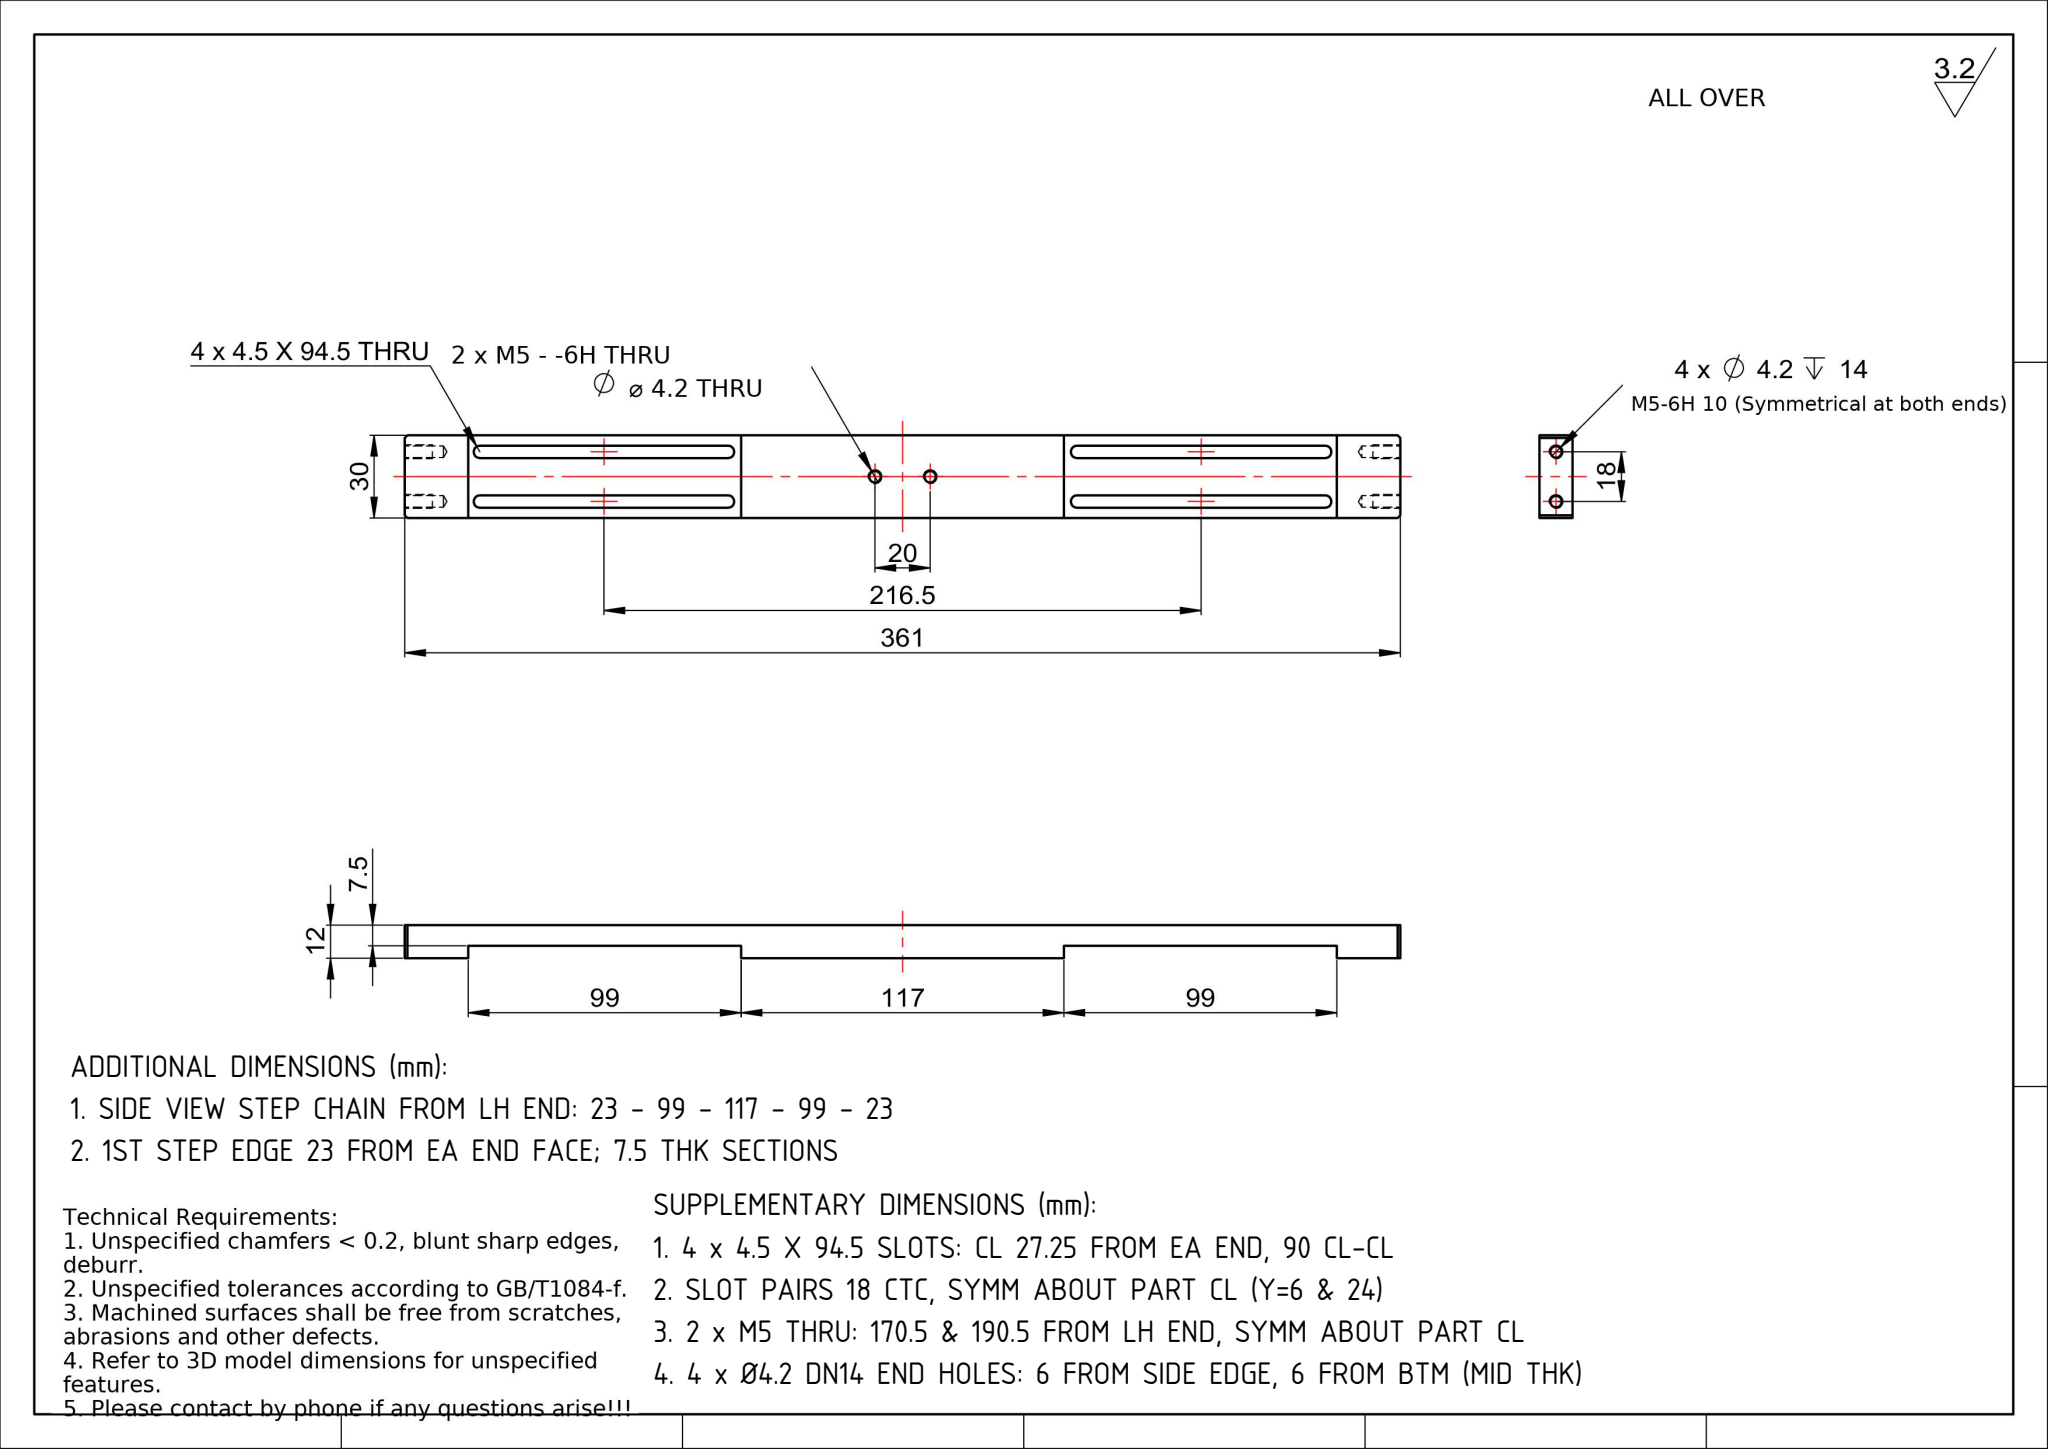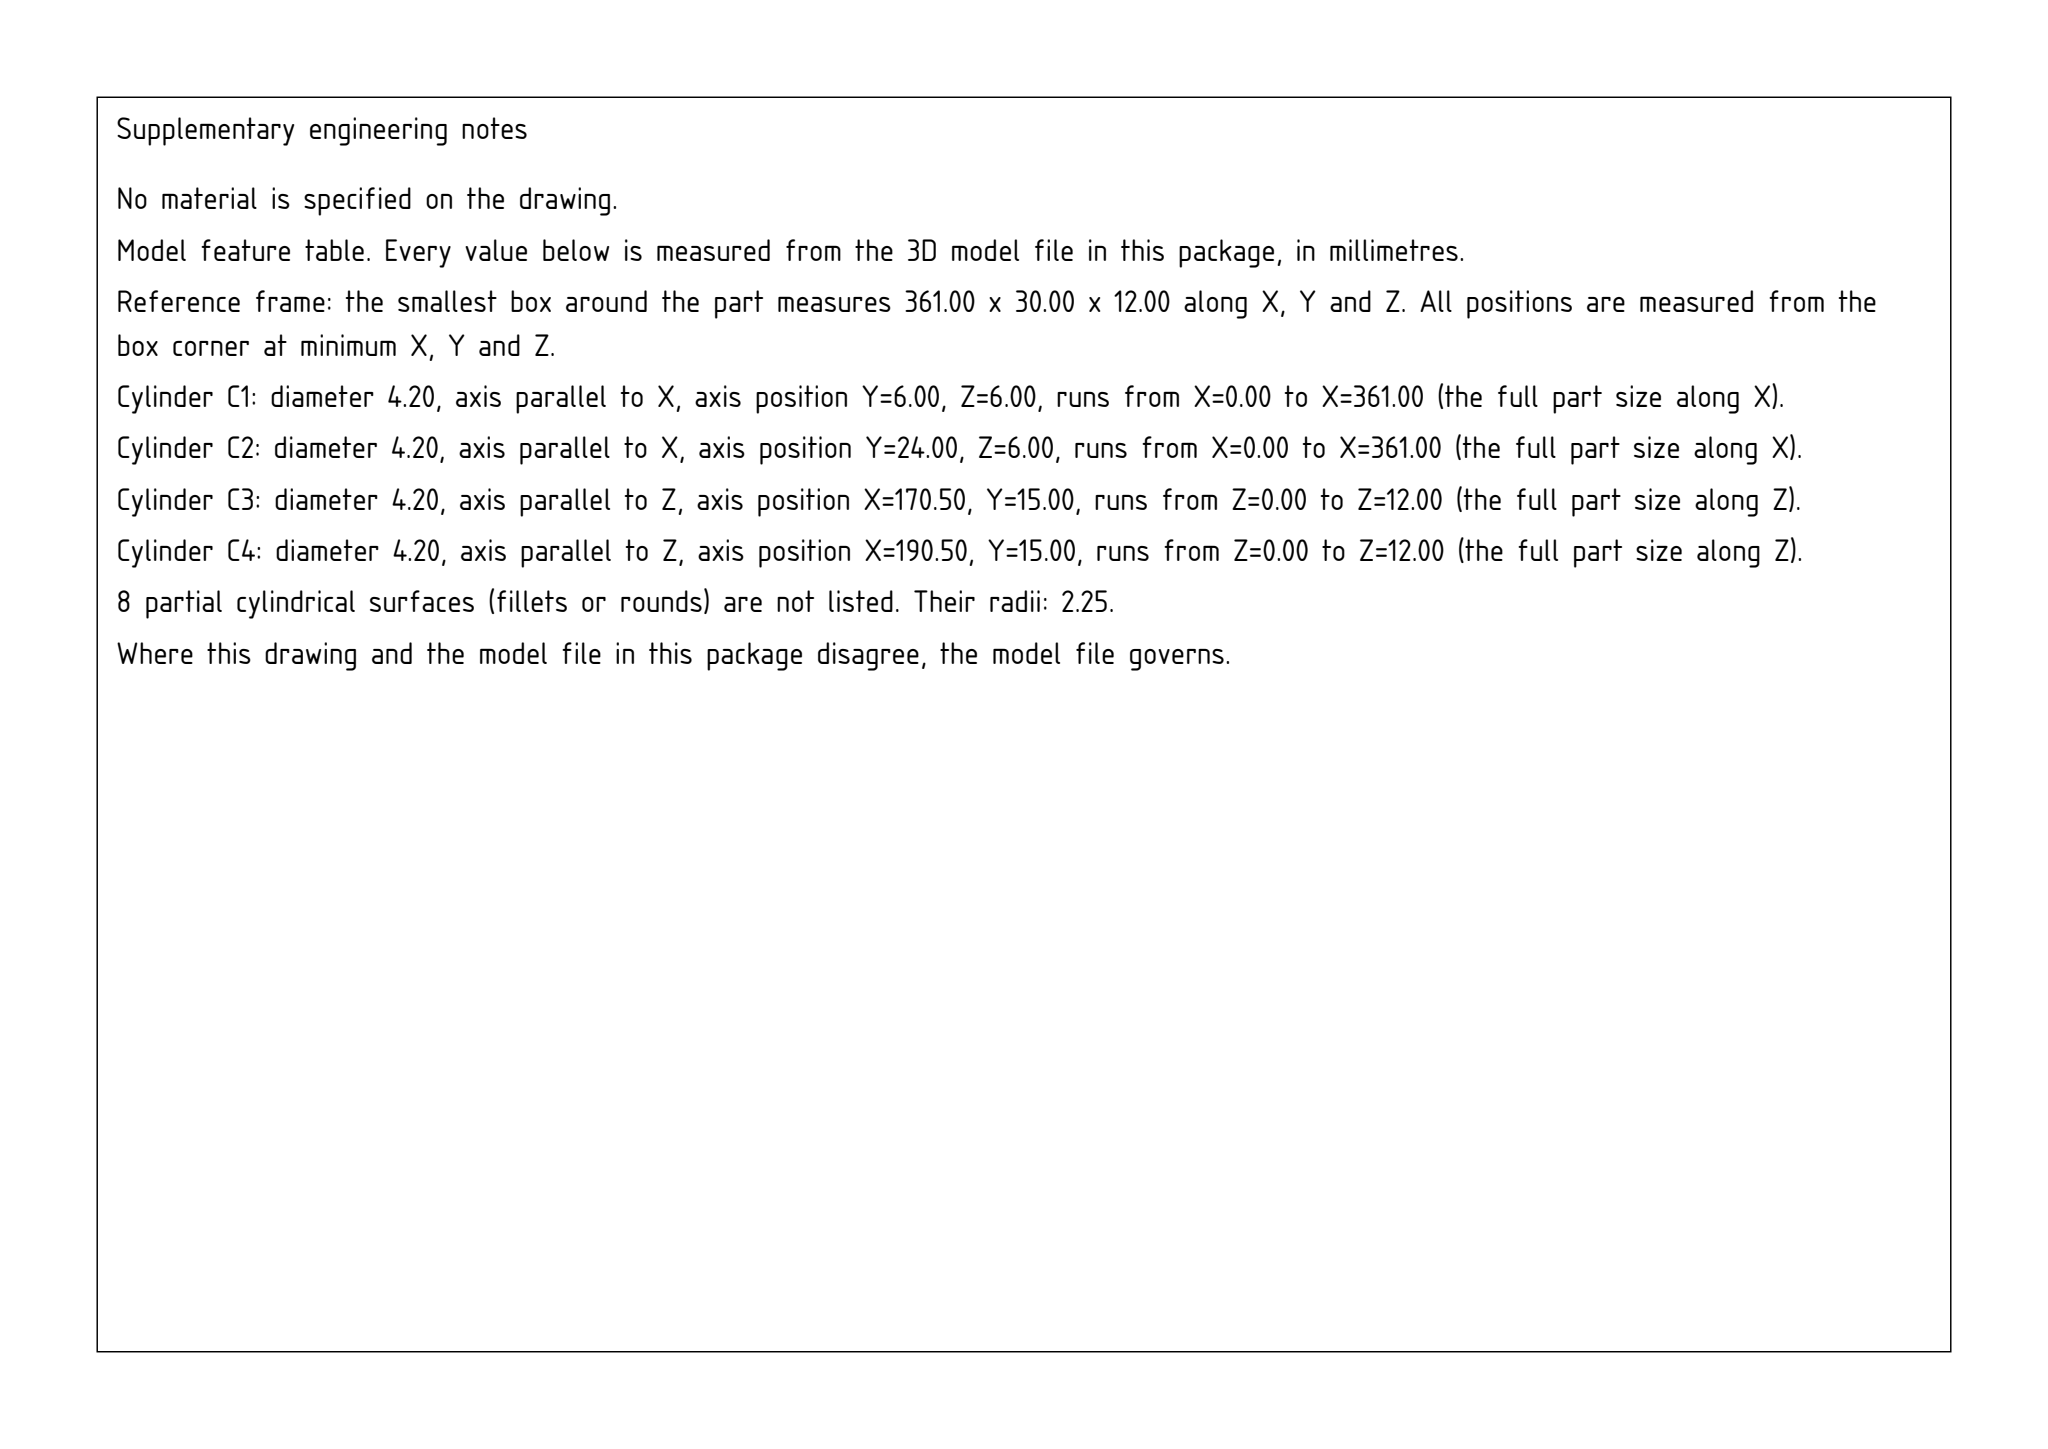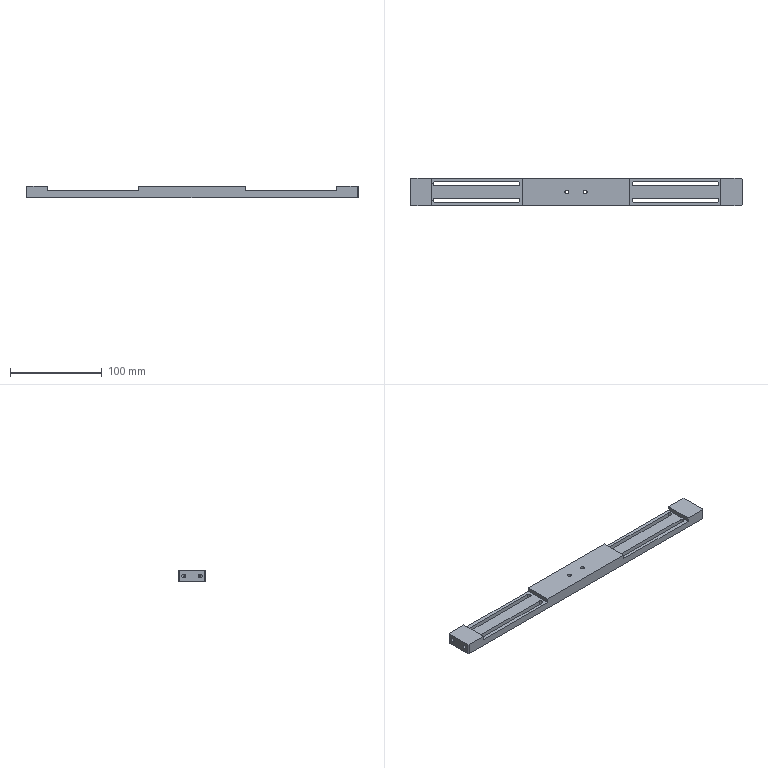Part | SolidWorks | mm | 1 solid | 58 faces | box 361 x 30 x 12 mm | volume 89447 mm3 | plane 26 | cylinder 24 | cone 8 | commonest cylinder face diameters 4.5 x12 4.2 x12
build123d program:
from build123d import *

# Parameters (mm, degrees)
SKETCH1_W                  = 361
SKETCH1_H                  = 30
BOSS_EXTRUDE1_DEPTH        = 6
M5_TAPPED_HOLE1_AT_2_COUNT = 2
M5_TAPPED_HOLE1_AT_2_PITCH = 18
SKETCH12_W                 = 99
SKETCH12_H                 = 30
CUT_EXTRUDE1_DEPTH         = 4.5
CUT_EXTRUDE2_DEPTH         = 182.519
CHAMFER1_SIZE              = 1
M5_TAPPED_HOLE2_D          = 4.2


with BuildPart() as part:
    # Sketch1 → Boss-Extrude1 (new, symmetric)
    with BuildSketch(Plane.XY):
        Rectangle(SKETCH1_W, SKETCH1_H)
    extrude(amount=BOSS_EXTRUDE1_DEPTH, both=True)

    # Sketch6 → M5 Tapped Hole1 (revolve, cut)
    with BuildSketch(Plane(origin=(-180.5, -9, 0), x_dir=(0, 0, 1), z_dir=(0, 1, 0))):
        Polygon((0, 0), (0, 15.262), (2.1, 14), (2.1, 0), align=None)
    m5_tapped_hole1 = revolve(axis=Axis((-186.85, -9, 0), (1, 0, 0)), mode=Mode.SUBTRACT)

    # M5 Tapped Hole1 at 2: M5 Tapped Hole1 ×2
    with Locations(*[(0, i * M5_TAPPED_HOLE1_AT_2_PITCH, 0) for i in range(1, M5_TAPPED_HOLE1_AT_2_COUNT)]):
        add(m5_tapped_hole1, mode=Mode.SUBTRACT)

    # Sketch12 → Cut-Extrude1 (cut)
    with BuildSketch(Plane.XY.offset(6)):
        with Locations((-108, 0)):
            Rectangle(SKETCH12_W, SKETCH12_H)
        with Locations((108, 0)):
            Rectangle(SKETCH12_W, SKETCH12_H)
    extrude(amount=-CUT_EXTRUDE1_DEPTH, mode=Mode.SUBTRACT)

    # Sketch8 → Cut-Extrude2 (cut, through all)
    with BuildSketch(Plane(origin=(0, 0, -6), x_dir=(-1, 0, 0), z_dir=(0, 0, -1))):
        with BuildLine():
            Line((153.25, -11.25), (63.25, -11.25))
            ThreePointArc((63.25, -11.25), (61, -9), (63.25, -6.75))
            Line((63.25, -6.75), (153.25, -6.75))
            ThreePointArc((153.25, -6.75), (155.5, -9), (153.25, -11.25))
        make_face()
        with BuildLine():
            Line((153.25, 6.75), (63.25, 6.75))
            ThreePointArc((63.25, 6.75), (61, 9), (63.25, 11.25))
            Line((63.25, 11.25), (153.25, 11.25))
            ThreePointArc((153.25, 11.25), (155.5, 9), (153.25, 6.75))
        make_face()
    cut_extrude2 = extrude(amount=-CUT_EXTRUDE2_DEPTH, mode=Mode.SUBTRACT)

    # Chamfer1
    chamfer1_edges = [part.edges().sort_by_distance(p)[0] for p in [
        (180.5, -15, 0),
        (-180.5, -15, 0),
        (-180.5, 15, 0),
        (180.5, 15, 0),
    ]]
    chamfer(chamfer1_edges, length=CHAMFER1_SIZE)

    # M5 Tapped Hole2 (through all)
    with Locations(Plane(origin=(0, 0, -6), x_dir=(-1, 0, 0), z_dir=(0, 0, -1))):
        with Locations((10, 0), (-10, 0)):
            Hole(M5_TAPPED_HOLE2_D / 2)

    # Mirror1: M5 Tapped Hole1, Cut-Extrude2 across plane
    add(m5_tapped_hole1.mirror(Plane(origin=(0, 0, 0), x_dir=(0, 0, 1), z_dir=(1, 0, 0))), mode=Mode.SUBTRACT)
    add(cut_extrude2.mirror(Plane(origin=(0, 0, 0), x_dir=(0, 0, 1), z_dir=(1, 0, 0))), mode=Mode.SUBTRACT)

    # Mirror1 copy 1 sketch → Mirror1 copy 1 (revolve, cut)
    with BuildSketch(Plane(origin=(180.5, 9, 0), x_dir=(0, 0, 1), z_dir=(0, 1, 0))):
        Polygon((0, 0), (0, -15.262), (2.1, -14), (2.1, 0), align=None)
    revolve(axis=Axis((186.85, 9, 0), (1, 0, 0)), mode=Mode.SUBTRACT)


solid = part.part